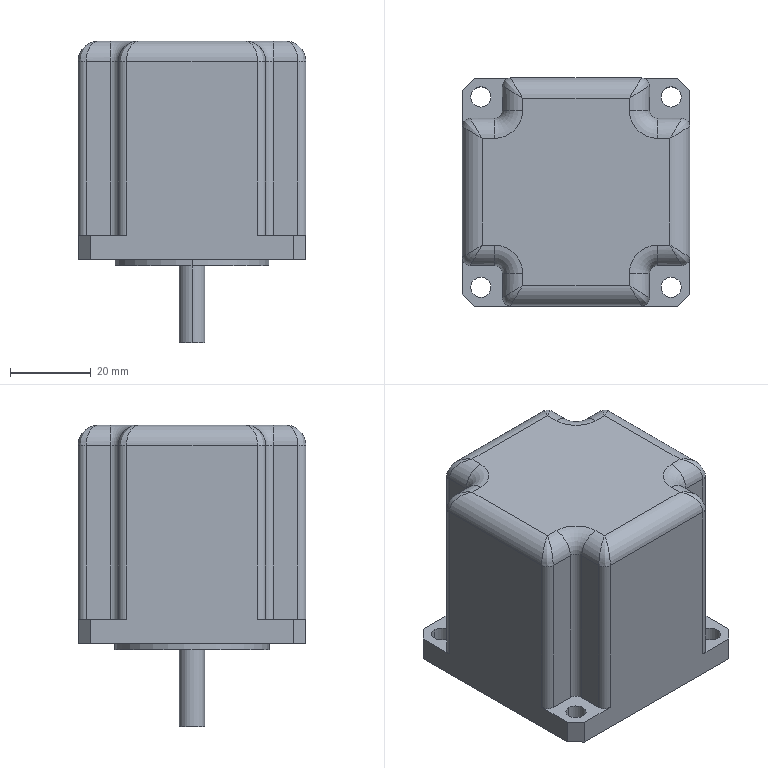Component | SolidWorks | SL010-RightStreamline-1-1_SL010-BeltMotorAssembly-1-1_SL010-LeadshineStepper-2-1-1 | 1 solid | 72 faces | volume 153132 mm3 | cylinder 36 | plane 24 | spline 8 | torus 4 | commonest cylinder face diameters 4 x12 10 x12 5 x8 6.35 x2 38.1 x2